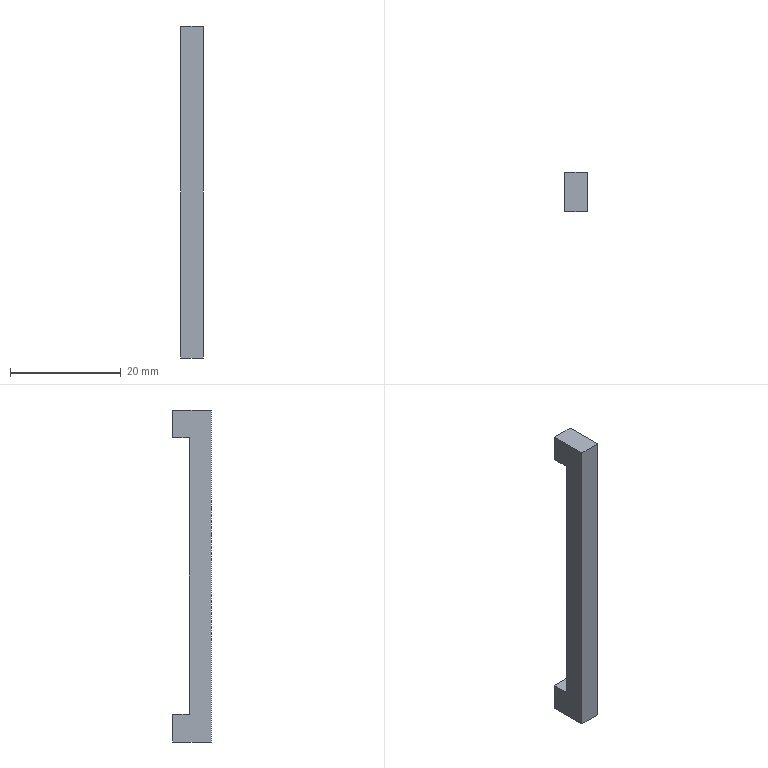Component | NX | KEY | 1 solid | 10 faces | box 4 x 7 x 60 mm | volume 1080 mm3 | plane 10
STEP:
#1=CARTESIAN_POINT('',(0.,0.,0.));
#2=DIRECTION('',(0.,0.,1.));
#3=DIRECTION('',(1.,0.,0.));
#4=AXIS2_PLACEMENT_3D('',#1,#2,#3);
#5=CARTESIAN_POINT('',(5.5,-11.365,13.5));
#6=VERTEX_POINT('',#5);
#7=CARTESIAN_POINT('',(5.5,-11.365,63.5));
#8=VERTEX_POINT('',#7);
#9=CARTESIAN_POINT('',(5.5,-11.365,38.5));
#10=DIRECTION('',(0.,0.,1.));
#11=VECTOR('',#10,1.);
#12=LINE('',#9,#11);
#13=CARTESIAN_POINT('',(9.5,-11.365,38.5));
#14=DIRECTION('',(0.,-1.,0.));
#15=DIRECTION('',(0.,-0.,-1.));
#16=AXIS2_PLACEMENT_3D('',#13,#14,#15);
#17=PLANE('',#16);
#18=CARTESIAN_POINT('',(0.,-4.));
#19=DIRECTION('',(-1.,0.));
#20=VECTOR('',#19,1.);
#21=LINE('',#18,#20);
#22=(GEOMETRIC_REPRESENTATION_CONTEXT(2)PARAMETRIC_REPRESENTATION_CONTEXT()REPRESENTATION_CONTEXT('',''));
#23=DEFINITIONAL_REPRESENTATION('',(#21),#22);
#24=PCURVE('',#17,#23);
#25=CARTESIAN_POINT('',(5.5,-11.365,38.5));
#26=DIRECTION('',(-1.,0.,0.));
#27=DIRECTION('',(0.,0.,1.));
#28=AXIS2_PLACEMENT_3D('',#25,#26,#27);
#29=PLANE('',#28);
#30=CARTESIAN_POINT('',(0.,0.));
#31=DIRECTION('',(1.,0.));
#32=VECTOR('',#31,1.);
#33=LINE('',#30,#32);
#34=(GEOMETRIC_REPRESENTATION_CONTEXT(2)PARAMETRIC_REPRESENTATION_CONTEXT()REPRESENTATION_CONTEXT('',''));
#35=DEFINITIONAL_REPRESENTATION('',(#33),#34);
#36=PCURVE('',#29,#35);
#37=SURFACE_CURVE('',#12,(#24,#36),.PCURVE_S1.);
#38=EDGE_CURVE('',#6,#8,#37,.T.);
#39=ORIENTED_EDGE('',*,*,#38,.T.);
#40=CARTESIAN_POINT('',(9.5,-11.365,63.5));
#41=VERTEX_POINT('',#40);
#42=CARTESIAN_POINT('',(9.5,-11.365,63.5));
#43=DIRECTION('',(-1.,0.,0.));
#44=VECTOR('',#43,1.);
#45=LINE('',#42,#44);
#46=CARTESIAN_POINT('',(-25.,0.));
#47=DIRECTION('',(0.,-1.));
#48=VECTOR('',#47,1.);
#49=LINE('',#46,#48);
#50=(GEOMETRIC_REPRESENTATION_CONTEXT(2)PARAMETRIC_REPRESENTATION_CONTEXT()REPRESENTATION_CONTEXT('',''));
#51=DEFINITIONAL_REPRESENTATION('',(#49),#50);
#52=PCURVE('',#17,#51);
#53=CARTESIAN_POINT('',(9.5,-11.365,63.5));
#54=DIRECTION('',(0.,0.,1.));
#55=DIRECTION('',(1.,0.,0.));
#56=AXIS2_PLACEMENT_3D('',#53,#54,#55);
#57=PLANE('',#56);
#58=CARTESIAN_POINT('',(0.,0.));
#59=DIRECTION('',(-1.,0.));
#60=VECTOR('',#59,1.);
#61=LINE('',#58,#60);
#62=(GEOMETRIC_REPRESENTATION_CONTEXT(2)PARAMETRIC_REPRESENTATION_CONTEXT()REPRESENTATION_CONTEXT('',''));
#63=DEFINITIONAL_REPRESENTATION('',(#61),#62);
#64=PCURVE('',#57,#63);
#65=SURFACE_CURVE('',#45,(#52,#64),.PCURVE_S1.);
#66=EDGE_CURVE('',#41,#8,#65,.T.);
#67=ORIENTED_EDGE('',*,*,#66,.F.);
#68=CARTESIAN_POINT('',(9.5,-11.365,13.5));
#69=VERTEX_POINT('',#68);
#70=CARTESIAN_POINT('',(9.5,-11.365,13.5));
#71=DIRECTION('',(0.,-0.,1.));
#72=VECTOR('',#71,1.);
#73=LINE('',#70,#72);
#74=CARTESIAN_POINT('',(25.,0.));
#75=DIRECTION('',(-1.,0.));
#76=VECTOR('',#75,1.);
#77=LINE('',#74,#76);
#78=(GEOMETRIC_REPRESENTATION_CONTEXT(2)PARAMETRIC_REPRESENTATION_CONTEXT()REPRESENTATION_CONTEXT('',''));
#79=DEFINITIONAL_REPRESENTATION('',(#77),#78);
#80=PCURVE('',#17,#79);
#81=CARTESIAN_POINT('',(9.5,-11.365,38.5));
#82=DIRECTION('',(-1.,0.,0.));
#83=DIRECTION('',(0.,0.,1.));
#84=AXIS2_PLACEMENT_3D('',#81,#82,#83);
#85=PLANE('',#84);
#86=CARTESIAN_POINT('',(-25.,0.));
#87=DIRECTION('',(1.,-0.));
#88=VECTOR('',#87,1.);
#89=LINE('',#86,#88);
#90=(GEOMETRIC_REPRESENTATION_CONTEXT(2)PARAMETRIC_REPRESENTATION_CONTEXT()REPRESENTATION_CONTEXT('',''));
#91=DEFINITIONAL_REPRESENTATION('',(#89),#90);
#92=PCURVE('',#85,#91);
#93=SURFACE_CURVE('',#73,(#80,#92),.PCURVE_S1.);
#94=EDGE_CURVE('',#69,#41,#93,.T.);
#95=ORIENTED_EDGE('',*,*,#94,.F.);
#96=CARTESIAN_POINT('',(9.5,-11.365,13.5));
#97=DIRECTION('',(-1.,0.,0.));
#98=VECTOR('',#97,1.);
#99=LINE('',#96,#98);
#100=CARTESIAN_POINT('',(25.,0.));
#101=DIRECTION('',(0.,-1.));
#102=VECTOR('',#101,1.);
#103=LINE('',#100,#102);
#104=(GEOMETRIC_REPRESENTATION_CONTEXT(2)PARAMETRIC_REPRESENTATION_CONTEXT()REPRESENTATION_CONTEXT('',''));
#105=DEFINITIONAL_REPRESENTATION('',(#103),#104);
#106=PCURVE('',#17,#105);
#107=CARTESIAN_POINT('',(9.5,-8.365,13.5));
#108=DIRECTION('',(0.,0.,-1.));
#109=DIRECTION('',(-1.,0.,0.));
#110=AXIS2_PLACEMENT_3D('',#107,#108,#109);
#111=PLANE('',#110);
#112=CARTESIAN_POINT('',(0.,-3.));
#113=DIRECTION('',(1.,0.));
#114=VECTOR('',#113,1.);
#115=LINE('',#112,#114);
#116=(GEOMETRIC_REPRESENTATION_CONTEXT(2)PARAMETRIC_REPRESENTATION_CONTEXT()REPRESENTATION_CONTEXT('',''));
#117=DEFINITIONAL_REPRESENTATION('',(#115),#116);
#118=PCURVE('',#111,#117);
#119=SURFACE_CURVE('',#99,(#106,#118),.PCURVE_S1.);
#120=EDGE_CURVE('',#69,#6,#119,.T.);
#121=ORIENTED_EDGE('',*,*,#120,.T.);
#122=EDGE_LOOP('',(#39,#67,#95,#121));
#123=FACE_BOUND('',#122,.T.);
#124=ADVANCED_FACE('',(#123),#17,.F.);
#125=CARTESIAN_POINT('',(5.5,-8.365,63.5));
#126=VERTEX_POINT('',#125);
#127=CARTESIAN_POINT('',(5.5,-11.365,63.5));
#128=DIRECTION('',(0.,1.,0.));
#129=VECTOR('',#128,1.);
#130=LINE('',#127,#129);
#131=CARTESIAN_POINT('',(-4.,0.));
#132=DIRECTION('',(0.,1.));
#133=VECTOR('',#132,1.);
#134=LINE('',#131,#133);
#135=(GEOMETRIC_REPRESENTATION_CONTEXT(2)PARAMETRIC_REPRESENTATION_CONTEXT()REPRESENTATION_CONTEXT('',''));
#136=DEFINITIONAL_REPRESENTATION('',(#134),#135);
#137=PCURVE('',#57,#136);
#138=CARTESIAN_POINT('',(25.,0.));
#139=DIRECTION('',(0.,1.));
#140=VECTOR('',#139,1.);
#141=LINE('',#138,#140);
#142=(GEOMETRIC_REPRESENTATION_CONTEXT(2)PARAMETRIC_REPRESENTATION_CONTEXT()REPRESENTATION_CONTEXT('',''));
#143=DEFINITIONAL_REPRESENTATION('',(#141),#142);
#144=PCURVE('',#29,#143);
#145=SURFACE_CURVE('',#130,(#137,#144),.PCURVE_S1.);
#146=EDGE_CURVE('',#8,#126,#145,.T.);
#147=ORIENTED_EDGE('',*,*,#146,.T.);
#148=CARTESIAN_POINT('',(9.5,-8.365,63.5));
#149=VERTEX_POINT('',#148);
#150=CARTESIAN_POINT('',(9.5,-8.365,63.5));
#151=DIRECTION('',(-1.,0.,0.));
#152=VECTOR('',#151,1.);
#153=LINE('',#150,#152);
#154=CARTESIAN_POINT('',(0.,3.));
#155=DIRECTION('',(-1.,0.));
#156=VECTOR('',#155,1.);
#157=LINE('',#154,#156);
#158=(GEOMETRIC_REPRESENTATION_CONTEXT(2)PARAMETRIC_REPRESENTATION_CONTEXT()REPRESENTATION_CONTEXT('',''));
#159=DEFINITIONAL_REPRESENTATION('',(#157),#158);
#160=PCURVE('',#57,#159);
#161=CARTESIAN_POINT('',(9.5,-8.365,63.5));
#162=DIRECTION('',(0.,-1.,0.));
#163=DIRECTION('',(0.,-0.,-1.));
#164=AXIS2_PLACEMENT_3D('',#161,#162,#163);
#165=PLANE('',#164);
#166=CARTESIAN_POINT('',(0.,0.));
#167=DIRECTION('',(0.,-1.));
#168=VECTOR('',#167,1.);
#169=LINE('',#166,#168);
#170=(GEOMETRIC_REPRESENTATION_CONTEXT(2)PARAMETRIC_REPRESENTATION_CONTEXT()REPRESENTATION_CONTEXT('',''));
#171=DEFINITIONAL_REPRESENTATION('',(#169),#170);
#172=PCURVE('',#165,#171);
#173=SURFACE_CURVE('',#153,(#160,#172),.PCURVE_S1.);
#174=EDGE_CURVE('',#149,#126,#173,.T.);
#175=ORIENTED_EDGE('',*,*,#174,.F.);
#176=CARTESIAN_POINT('',(9.5,-11.365,63.5));
#177=DIRECTION('',(0.,1.,0.));
#178=VECTOR('',#177,1.);
#179=LINE('',#176,#178);
#180=CARTESIAN_POINT('',(0.,0.));
#181=DIRECTION('',(0.,1.));
#182=VECTOR('',#181,1.);
#183=LINE('',#180,#182);
#184=(GEOMETRIC_REPRESENTATION_CONTEXT(2)PARAMETRIC_REPRESENTATION_CONTEXT()REPRESENTATION_CONTEXT('',''));
#185=DEFINITIONAL_REPRESENTATION('',(#183),#184);
#186=PCURVE('',#57,#185);
#187=CARTESIAN_POINT('',(25.,0.));
#188=DIRECTION('',(0.,1.));
#189=VECTOR('',#188,1.);
#190=LINE('',#187,#189);
#191=(GEOMETRIC_REPRESENTATION_CONTEXT(2)PARAMETRIC_REPRESENTATION_CONTEXT()REPRESENTATION_CONTEXT('',''));
#192=DEFINITIONAL_REPRESENTATION('',(#190),#191);
#193=PCURVE('',#85,#192);
#194=SURFACE_CURVE('',#179,(#186,#193),.PCURVE_S1.);
#195=EDGE_CURVE('',#41,#149,#194,.T.);
#196=ORIENTED_EDGE('',*,*,#195,.F.);
#197=ORIENTED_EDGE('',*,*,#66,.T.);
#198=EDGE_LOOP('',(#147,#175,#196,#197));
#199=FACE_BOUND('',#198,.T.);
#200=ADVANCED_FACE('',(#199),#57,.F.);
#201=CARTESIAN_POINT('',(5.5,-8.365,68.5));
#202=VERTEX_POINT('',#201);
#203=CARTESIAN_POINT('',(5.5,-8.365,63.5));
#204=DIRECTION('',(0.,0.,1.));
#205=VECTOR('',#204,1.);
#206=LINE('',#203,#205);
#207=CARTESIAN_POINT('',(0.,-4.));
#208=DIRECTION('',(-1.,0.));
#209=VECTOR('',#208,1.);
#210=LINE('',#207,#209);
#211=(GEOMETRIC_REPRESENTATION_CONTEXT(2)PARAMETRIC_REPRESENTATION_CONTEXT()REPRESENTATION_CONTEXT('',''));
#212=DEFINITIONAL_REPRESENTATION('',(#210),#211);
#213=PCURVE('',#165,#212);
#214=CARTESIAN_POINT('',(25.,3.));
#215=DIRECTION('',(1.,0.));
#216=VECTOR('',#215,1.);
#217=LINE('',#214,#216);
#218=(GEOMETRIC_REPRESENTATION_CONTEXT(2)PARAMETRIC_REPRESENTATION_CONTEXT()REPRESENTATION_CONTEXT('',''));
#219=DEFINITIONAL_REPRESENTATION('',(#217),#218);
#220=PCURVE('',#29,#219);
#221=SURFACE_CURVE('',#206,(#213,#220),.PCURVE_S1.);
#222=EDGE_CURVE('',#126,#202,#221,.T.);
#223=ORIENTED_EDGE('',*,*,#222,.T.);
#224=CARTESIAN_POINT('',(9.5,-8.365,68.5));
#225=VERTEX_POINT('',#224);
#226=CARTESIAN_POINT('',(9.5,-8.365,68.5));
#227=DIRECTION('',(-1.,0.,0.));
#228=VECTOR('',#227,1.);
#229=LINE('',#226,#228);
#230=CARTESIAN_POINT('',(-5.,0.));
#231=DIRECTION('',(0.,-1.));
#232=VECTOR('',#231,1.);
#233=LINE('',#230,#232);
#234=(GEOMETRIC_REPRESENTATION_CONTEXT(2)PARAMETRIC_REPRESENTATION_CONTEXT()REPRESENTATION_CONTEXT('',''));
#235=DEFINITIONAL_REPRESENTATION('',(#233),#234);
#236=PCURVE('',#165,#235);
#237=CARTESIAN_POINT('',(9.5,-8.365,68.5));
#238=DIRECTION('',(0.,0.,-1.));
#239=DIRECTION('',(-1.,0.,0.));
#240=AXIS2_PLACEMENT_3D('',#237,#238,#239);
#241=PLANE('',#240);
#242=CARTESIAN_POINT('',(0.,0.));
#243=DIRECTION('',(1.,0.));
#244=VECTOR('',#243,1.);
#245=LINE('',#242,#244);
#246=(GEOMETRIC_REPRESENTATION_CONTEXT(2)PARAMETRIC_REPRESENTATION_CONTEXT()REPRESENTATION_CONTEXT('',''));
#247=DEFINITIONAL_REPRESENTATION('',(#245),#246);
#248=PCURVE('',#241,#247);
#249=SURFACE_CURVE('',#229,(#236,#248),.PCURVE_S1.);
#250=EDGE_CURVE('',#225,#202,#249,.T.);
#251=ORIENTED_EDGE('',*,*,#250,.F.);
#252=CARTESIAN_POINT('',(9.5,-8.365,63.5));
#253=DIRECTION('',(0.,0.,1.));
#254=VECTOR('',#253,1.);
#255=LINE('',#252,#254);
#256=CARTESIAN_POINT('',(0.,0.));
#257=DIRECTION('',(-1.,0.));
#258=VECTOR('',#257,1.);
#259=LINE('',#256,#258);
#260=(GEOMETRIC_REPRESENTATION_CONTEXT(2)PARAMETRIC_REPRESENTATION_CONTEXT()REPRESENTATION_CONTEXT('',''));
#261=DEFINITIONAL_REPRESENTATION('',(#259),#260);
#262=PCURVE('',#165,#261);
#263=CARTESIAN_POINT('',(25.,3.));
#264=DIRECTION('',(1.,0.));
#265=VECTOR('',#264,1.);
#266=LINE('',#263,#265);
#267=(GEOMETRIC_REPRESENTATION_CONTEXT(2)PARAMETRIC_REPRESENTATION_CONTEXT()REPRESENTATION_CONTEXT('',''));
#268=DEFINITIONAL_REPRESENTATION('',(#266),#267);
#269=PCURVE('',#85,#268);
#270=SURFACE_CURVE('',#255,(#262,#269),.PCURVE_S1.);
#271=EDGE_CURVE('',#149,#225,#270,.T.);
#272=ORIENTED_EDGE('',*,*,#271,.F.);
#273=ORIENTED_EDGE('',*,*,#174,.T.);
#274=EDGE_LOOP('',(#223,#251,#272,#273));
#275=FACE_BOUND('',#274,.T.);
#276=ADVANCED_FACE('',(#275),#165,.F.);
#277=CARTESIAN_POINT('',(5.5,-15.365,68.5));
#278=VERTEX_POINT('',#277);
#279=CARTESIAN_POINT('',(5.5,-8.365,68.5));
#280=DIRECTION('',(0.,-1.,0.));
#281=VECTOR('',#280,1.);
#282=LINE('',#279,#281);
#283=CARTESIAN_POINT('',(4.,0.));
#284=DIRECTION('',(0.,-1.));
#285=VECTOR('',#284,1.);
#286=LINE('',#283,#285);
#287=(GEOMETRIC_REPRESENTATION_CONTEXT(2)PARAMETRIC_REPRESENTATION_CONTEXT()REPRESENTATION_CONTEXT('',''));
#288=DEFINITIONAL_REPRESENTATION('',(#286),#287);
#289=PCURVE('',#241,#288);
#290=CARTESIAN_POINT('',(30.,3.));
#291=DIRECTION('',(0.,-1.));
#292=VECTOR('',#291,1.);
#293=LINE('',#290,#292);
#294=(GEOMETRIC_REPRESENTATION_CONTEXT(2)PARAMETRIC_REPRESENTATION_CONTEXT()REPRESENTATION_CONTEXT('',''));
#295=DEFINITIONAL_REPRESENTATION('',(#293),#294);
#296=PCURVE('',#29,#295);
#297=SURFACE_CURVE('',#282,(#289,#296),.PCURVE_S1.);
#298=EDGE_CURVE('',#202,#278,#297,.T.);
#299=ORIENTED_EDGE('',*,*,#298,.T.);
#300=CARTESIAN_POINT('',(9.5,-15.365,68.5));
#301=VERTEX_POINT('',#300);
#302=CARTESIAN_POINT('',(9.5,-15.365,68.5));
#303=DIRECTION('',(-1.,0.,0.));
#304=VECTOR('',#303,1.);
#305=LINE('',#302,#304);
#306=CARTESIAN_POINT('',(0.,-7.));
#307=DIRECTION('',(1.,0.));
#308=VECTOR('',#307,1.);
#309=LINE('',#306,#308);
#310=(GEOMETRIC_REPRESENTATION_CONTEXT(2)PARAMETRIC_REPRESENTATION_CONTEXT()REPRESENTATION_CONTEXT('',''));
#311=DEFINITIONAL_REPRESENTATION('',(#309),#310);
#312=PCURVE('',#241,#311);
#313=CARTESIAN_POINT('',(9.5,-15.365,38.5));
#314=DIRECTION('',(0.,1.,0.));
#315=DIRECTION('',(0.,-0.,1.));
#316=AXIS2_PLACEMENT_3D('',#313,#314,#315);
#317=PLANE('',#316);
#318=CARTESIAN_POINT('',(30.,0.));
#319=DIRECTION('',(0.,-1.));
#320=VECTOR('',#319,1.);
#321=LINE('',#318,#320);
#322=(GEOMETRIC_REPRESENTATION_CONTEXT(2)PARAMETRIC_REPRESENTATION_CONTEXT()REPRESENTATION_CONTEXT('',''));
#323=DEFINITIONAL_REPRESENTATION('',(#321),#322);
#324=PCURVE('',#317,#323);
#325=SURFACE_CURVE('',#305,(#312,#324),.PCURVE_S1.);
#326=EDGE_CURVE('',#301,#278,#325,.T.);
#327=ORIENTED_EDGE('',*,*,#326,.F.);
#328=CARTESIAN_POINT('',(9.5,-8.365,68.5));
#329=DIRECTION('',(0.,-1.,0.));
#330=VECTOR('',#329,1.);
#331=LINE('',#328,#330);
#332=CARTESIAN_POINT('',(0.,0.));
#333=DIRECTION('',(0.,-1.));
#334=VECTOR('',#333,1.);
#335=LINE('',#332,#334);
#336=(GEOMETRIC_REPRESENTATION_CONTEXT(2)PARAMETRIC_REPRESENTATION_CONTEXT()REPRESENTATION_CONTEXT('',''));
#337=DEFINITIONAL_REPRESENTATION('',(#335),#336);
#338=PCURVE('',#241,#337);
#339=CARTESIAN_POINT('',(30.,3.));
#340=DIRECTION('',(0.,-1.));
#341=VECTOR('',#340,1.);
#342=LINE('',#339,#341);
#343=(GEOMETRIC_REPRESENTATION_CONTEXT(2)PARAMETRIC_REPRESENTATION_CONTEXT()REPRESENTATION_CONTEXT('',''));
#344=DEFINITIONAL_REPRESENTATION('',(#342),#343);
#345=PCURVE('',#85,#344);
#346=SURFACE_CURVE('',#331,(#338,#345),.PCURVE_S1.);
#347=EDGE_CURVE('',#225,#301,#346,.T.);
#348=ORIENTED_EDGE('',*,*,#347,.F.);
#349=ORIENTED_EDGE('',*,*,#250,.T.);
#350=EDGE_LOOP('',(#299,#327,#348,#349));
#351=FACE_BOUND('',#350,.T.);
#352=ADVANCED_FACE('',(#351),#241,.F.);
#353=CARTESIAN_POINT('',(5.5,-15.365,8.5));
#354=VERTEX_POINT('',#353);
#355=CARTESIAN_POINT('',(5.5,-15.365,38.5));
#356=DIRECTION('',(0.,0.,-1.));
#357=VECTOR('',#356,1.);
#358=LINE('',#355,#357);
#359=CARTESIAN_POINT('',(0.,-4.));
#360=DIRECTION('',(-1.,0.));
#361=VECTOR('',#360,1.);
#362=LINE('',#359,#361);
#363=(GEOMETRIC_REPRESENTATION_CONTEXT(2)PARAMETRIC_REPRESENTATION_CONTEXT()REPRESENTATION_CONTEXT('',''));
#364=DEFINITIONAL_REPRESENTATION('',(#362),#363);
#365=PCURVE('',#317,#364);
#366=CARTESIAN_POINT('',(0.,-4.));
#367=DIRECTION('',(-1.,0.));
#368=VECTOR('',#367,1.);
#369=LINE('',#366,#368);
#370=(GEOMETRIC_REPRESENTATION_CONTEXT(2)PARAMETRIC_REPRESENTATION_CONTEXT()REPRESENTATION_CONTEXT('',''));
#371=DEFINITIONAL_REPRESENTATION('',(#369),#370);
#372=PCURVE('',#29,#371);
#373=SURFACE_CURVE('',#358,(#365,#372),.PCURVE_S1.);
#374=EDGE_CURVE('',#278,#354,#373,.T.);
#375=ORIENTED_EDGE('',*,*,#374,.T.);
#376=CARTESIAN_POINT('',(9.5,-15.365,8.5));
#377=VERTEX_POINT('',#376);
#378=CARTESIAN_POINT('',(9.5,-15.365,8.5));
#379=DIRECTION('',(-1.,0.,0.));
#380=VECTOR('',#379,1.);
#381=LINE('',#378,#380);
#382=CARTESIAN_POINT('',(-30.,0.));
#383=DIRECTION('',(0.,-1.));
#384=VECTOR('',#383,1.);
#385=LINE('',#382,#384);
#386=(GEOMETRIC_REPRESENTATION_CONTEXT(2)PARAMETRIC_REPRESENTATION_CONTEXT()REPRESENTATION_CONTEXT('',''));
#387=DEFINITIONAL_REPRESENTATION('',(#385),#386);
#388=PCURVE('',#317,#387);
#389=CARTESIAN_POINT('',(9.5,-15.365,8.5));
#390=DIRECTION('',(0.,0.,1.));
#391=DIRECTION('',(1.,0.,0.));
#392=AXIS2_PLACEMENT_3D('',#389,#390,#391);
#393=PLANE('',#392);
#394=CARTESIAN_POINT('',(0.,0.));
#395=DIRECTION('',(-1.,0.));
#396=VECTOR('',#395,1.);
#397=LINE('',#394,#396);
#398=(GEOMETRIC_REPRESENTATION_CONTEXT(2)PARAMETRIC_REPRESENTATION_CONTEXT()REPRESENTATION_CONTEXT('',''));
#399=DEFINITIONAL_REPRESENTATION('',(#397),#398);
#400=PCURVE('',#393,#399);
#401=SURFACE_CURVE('',#381,(#388,#400),.PCURVE_S1.);
#402=EDGE_CURVE('',#377,#354,#401,.T.);
#403=ORIENTED_EDGE('',*,*,#402,.F.);
#404=CARTESIAN_POINT('',(9.5,-15.365,68.5));
#405=DIRECTION('',(0.,-0.,-1.));
#406=VECTOR('',#405,1.);
#407=LINE('',#404,#406);
#408=CARTESIAN_POINT('',(30.,0.));
#409=DIRECTION('',(-1.,0.));
#410=VECTOR('',#409,1.);
#411=LINE('',#408,#410);
#412=(GEOMETRIC_REPRESENTATION_CONTEXT(2)PARAMETRIC_REPRESENTATION_CONTEXT()REPRESENTATION_CONTEXT('',''));
#413=DEFINITIONAL_REPRESENTATION('',(#411),#412);
#414=PCURVE('',#317,#413);
#415=CARTESIAN_POINT('',(30.,-4.));
#416=DIRECTION('',(-1.,-0.));
#417=VECTOR('',#416,1.);
#418=LINE('',#415,#417);
#419=(GEOMETRIC_REPRESENTATION_CONTEXT(2)PARAMETRIC_REPRESENTATION_CONTEXT()REPRESENTATION_CONTEXT('',''));
#420=DEFINITIONAL_REPRESENTATION('',(#418),#419);
#421=PCURVE('',#85,#420);
#422=SURFACE_CURVE('',#407,(#414,#421),.PCURVE_S1.);
#423=EDGE_CURVE('',#301,#377,#422,.T.);
#424=ORIENTED_EDGE('',*,*,#423,.F.);
#425=ORIENTED_EDGE('',*,*,#326,.T.);
#426=EDGE_LOOP('',(#375,#403,#424,#425));
#427=FACE_BOUND('',#426,.T.);
#428=ADVANCED_FACE('',(#427),#317,.F.);
#429=CARTESIAN_POINT('',(5.5,-8.365,8.5));
#430=VERTEX_POINT('',#429);
#431=CARTESIAN_POINT('',(5.5,-15.365,8.5));
#432=DIRECTION('',(0.,1.,0.));
#433=VECTOR('',#432,1.);
#434=LINE('',#431,#433);
#435=CARTESIAN_POINT('',(-4.,0.));
#436=DIRECTION('',(0.,1.));
#437=VECTOR('',#436,1.);
#438=LINE('',#435,#437);
#439=(GEOMETRIC_REPRESENTATION_CONTEXT(2)PARAMETRIC_REPRESENTATION_CONTEXT()REPRESENTATION_CONTEXT('',''));
#440=DEFINITIONAL_REPRESENTATION('',(#438),#439);
#441=PCURVE('',#393,#440);
#442=CARTESIAN_POINT('',(-30.,-4.));
#443=DIRECTION('',(0.,1.));
#444=VECTOR('',#443,1.);
#445=LINE('',#442,#444);
#446=(GEOMETRIC_REPRESENTATION_CONTEXT(2)PARAMETRIC_REPRESENTATION_CONTEXT()REPRESENTATION_CONTEXT('',''));
#447=DEFINITIONAL_REPRESENTATION('',(#445),#446);
#448=PCURVE('',#29,#447);
#449=SURFACE_CURVE('',#434,(#441,#448),.PCURVE_S1.);
#450=EDGE_CURVE('',#354,#430,#449,.T.);
#451=ORIENTED_EDGE('',*,*,#450,.T.);
#452=CARTESIAN_POINT('',(9.5,-8.365,8.5));
#453=VERTEX_POINT('',#452);
#454=CARTESIAN_POINT('',(9.5,-8.365,8.5));
#455=DIRECTION('',(-1.,0.,0.));
#456=VECTOR('',#455,1.);
#457=LINE('',#454,#456);
#458=CARTESIAN_POINT('',(0.,7.));
#459=DIRECTION('',(-1.,0.));
#460=VECTOR('',#459,1.);
#461=LINE('',#458,#460);
#462=(GEOMETRIC_REPRESENTATION_CONTEXT(2)PARAMETRIC_REPRESENTATION_CONTEXT()REPRESENTATION_CONTEXT('',''));
#463=DEFINITIONAL_REPRESENTATION('',(#461),#462);
#464=PCURVE('',#393,#463);
#465=CARTESIAN_POINT('',(9.5,-8.365,8.5));
#466=DIRECTION('',(0.,-1.,-0.));
#467=DIRECTION('',(0.,0.,-1.));
#468=AXIS2_PLACEMENT_3D('',#465,#466,#467);
#469=PLANE('',#468);
#470=CARTESIAN_POINT('',(0.,0.));
#471=DIRECTION('',(0.,-1.));
#472=VECTOR('',#471,1.);
#473=LINE('',#470,#472);
#474=(GEOMETRIC_REPRESENTATION_CONTEXT(2)PARAMETRIC_REPRESENTATION_CONTEXT()REPRESENTATION_CONTEXT('',''));
#475=DEFINITIONAL_REPRESENTATION('',(#473),#474);
#476=PCURVE('',#469,#475);
#477=SURFACE_CURVE('',#457,(#464,#476),.PCURVE_S1.);
#478=EDGE_CURVE('',#453,#430,#477,.T.);
#479=ORIENTED_EDGE('',*,*,#478,.F.);
#480=CARTESIAN_POINT('',(9.5,-15.365,8.5));
#481=DIRECTION('',(0.,1.,0.));
#482=VECTOR('',#481,1.);
#483=LINE('',#480,#482);
#484=CARTESIAN_POINT('',(0.,0.));
#485=DIRECTION('',(0.,1.));
#486=VECTOR('',#485,1.);
#487=LINE('',#484,#486);
#488=(GEOMETRIC_REPRESENTATION_CONTEXT(2)PARAMETRIC_REPRESENTATION_CONTEXT()REPRESENTATION_CONTEXT('',''));
#489=DEFINITIONAL_REPRESENTATION('',(#487),#488);
#490=PCURVE('',#393,#489);
#491=CARTESIAN_POINT('',(-30.,-4.));
#492=DIRECTION('',(0.,1.));
#493=VECTOR('',#492,1.);
#494=LINE('',#491,#493);
#495=(GEOMETRIC_REPRESENTATION_CONTEXT(2)PARAMETRIC_REPRESENTATION_CONTEXT()REPRESENTATION_CONTEXT('',''));
#496=DEFINITIONAL_REPRESENTATION('',(#494),#495);
#497=PCURVE('',#85,#496);
#498=SURFACE_CURVE('',#483,(#490,#497),.PCURVE_S1.);
#499=EDGE_CURVE('',#377,#453,#498,.T.);
#500=ORIENTED_EDGE('',*,*,#499,.F.);
#501=ORIENTED_EDGE('',*,*,#402,.T.);
#502=EDGE_LOOP('',(#451,#479,#500,#501));
#503=FACE_BOUND('',#502,.T.);
#504=ADVANCED_FACE('',(#503),#393,.F.);
#505=CARTESIAN_POINT('',(5.5,-8.365,13.5));
#506=VERTEX_POINT('',#505);
#507=CARTESIAN_POINT('',(5.5,-8.365,8.5));
#508=DIRECTION('',(0.,-0.,1.));
#509=VECTOR('',#508,1.);
#510=LINE('',#507,#509);
#511=CARTESIAN_POINT('',(0.,-4.));
#512=DIRECTION('',(-1.,0.));
#513=VECTOR('',#512,1.);
#514=LINE('',#511,#513);
#515=(GEOMETRIC_REPRESENTATION_CONTEXT(2)PARAMETRIC_REPRESENTATION_CONTEXT()REPRESENTATION_CONTEXT('',''));
#516=DEFINITIONAL_REPRESENTATION('',(#514),#515);
#517=PCURVE('',#469,#516);
#518=CARTESIAN_POINT('',(-30.,3.));
#519=DIRECTION('',(1.,-0.));
#520=VECTOR('',#519,1.);
#521=LINE('',#518,#520);
#522=(GEOMETRIC_REPRESENTATION_CONTEXT(2)PARAMETRIC_REPRESENTATION_CONTEXT()REPRESENTATION_CONTEXT('',''));
#523=DEFINITIONAL_REPRESENTATION('',(#521),#522);
#524=PCURVE('',#29,#523);
#525=SURFACE_CURVE('',#510,(#517,#524),.PCURVE_S1.);
#526=EDGE_CURVE('',#430,#506,#525,.T.);
#527=ORIENTED_EDGE('',*,*,#526,.T.);
#528=CARTESIAN_POINT('',(9.5,-8.365,13.5));
#529=VERTEX_POINT('',#528);
#530=CARTESIAN_POINT('',(9.5,-8.365,13.5));
#531=DIRECTION('',(-1.,0.,0.));
#532=VECTOR('',#531,1.);
#533=LINE('',#530,#532);
#534=CARTESIAN_POINT('',(-5.,0.));
#535=DIRECTION('',(0.,-1.));
#536=VECTOR('',#535,1.);
#537=LINE('',#534,#536);
#538=(GEOMETRIC_REPRESENTATION_CONTEXT(2)PARAMETRIC_REPRESENTATION_CONTEXT()REPRESENTATION_CONTEXT('',''));
#539=DEFINITIONAL_REPRESENTATION('',(#537),#538);
#540=PCURVE('',#469,#539);
#541=CARTESIAN_POINT('',(0.,0.));
#542=DIRECTION('',(1.,0.));
#543=VECTOR('',#542,1.);
#544=LINE('',#541,#543);
#545=(GEOMETRIC_REPRESENTATION_CONTEXT(2)PARAMETRIC_REPRESENTATION_CONTEXT()REPRESENTATION_CONTEXT('',''));
#546=DEFINITIONAL_REPRESENTATION('',(#544),#545);
#547=PCURVE('',#111,#546);
#548=SURFACE_CURVE('',#533,(#540,#547),.PCURVE_S1.);
#549=EDGE_CURVE('',#529,#506,#548,.T.);
#550=ORIENTED_EDGE('',*,*,#549,.F.);
#551=CARTESIAN_POINT('',(9.5,-8.365,8.5));
#552=DIRECTION('',(0.,-0.,1.));
#553=VECTOR('',#552,1.);
#554=LINE('',#551,#553);
#555=CARTESIAN_POINT('',(0.,0.));
#556=DIRECTION('',(-1.,0.));
#557=VECTOR('',#556,1.);
#558=LINE('',#555,#557);
#559=(GEOMETRIC_REPRESENTATION_CONTEXT(2)PARAMETRIC_REPRESENTATION_CONTEXT()REPRESENTATION_CONTEXT('',''));
#560=DEFINITIONAL_REPRESENTATION('',(#558),#559);
#561=PCURVE('',#469,#560);
#562=CARTESIAN_POINT('',(-30.,3.));
#563=DIRECTION('',(1.,-0.));
#564=VECTOR('',#563,1.);
#565=LINE('',#562,#564);
#566=(GEOMETRIC_REPRESENTATION_CONTEXT(2)PARAMETRIC_REPRESENTATION_CONTEXT()REPRESENTATION_CONTEXT('',''));
#567=DEFINITIONAL_REPRESENTATION('',(#565),#566);
#568=PCURVE('',#85,#567);
#569=SURFACE_CURVE('',#554,(#561,#568),.PCURVE_S1.);
#570=EDGE_CURVE('',#453,#529,#569,.T.);
#571=ORIENTED_EDGE('',*,*,#570,.F.);
#572=ORIENTED_EDGE('',*,*,#478,.T.);
#573=EDGE_LOOP('',(#527,#550,#571,#572));
#574=FACE_BOUND('',#573,.T.);
#575=ADVANCED_FACE('',(#574),#469,.F.);
#576=CARTESIAN_POINT('',(5.5,-8.365,13.5));
#577=DIRECTION('',(0.,-1.,0.));
#578=VECTOR('',#577,1.);
#579=LINE('',#576,#578);
#580=CARTESIAN_POINT('',(4.,0.));
#581=DIRECTION('',(0.,-1.));
#582=VECTOR('',#581,1.);
#583=LINE('',#580,#582);
#584=(GEOMETRIC_REPRESENTATION_CONTEXT(2)PARAMETRIC_REPRESENTATION_CONTEXT()REPRESENTATION_CONTEXT('',''));
#585=DEFINITIONAL_REPRESENTATION('',(#583),#584);
#586=PCURVE('',#111,#585);
#587=CARTESIAN_POINT('',(-25.,3.));
#588=DIRECTION('',(0.,-1.));
#589=VECTOR('',#588,1.);
#590=LINE('',#587,#589);
#591=(GEOMETRIC_REPRESENTATION_CONTEXT(2)PARAMETRIC_REPRESENTATION_CONTEXT()REPRESENTATION_CONTEXT('',''));
#592=DEFINITIONAL_REPRESENTATION('',(#590),#591);
#593=PCURVE('',#29,#592);
#594=SURFACE_CURVE('',#579,(#586,#593),.PCURVE_S1.);
#595=EDGE_CURVE('',#506,#6,#594,.T.);
#596=ORIENTED_EDGE('',*,*,#595,.T.);
#597=ORIENTED_EDGE('',*,*,#120,.F.);
#598=CARTESIAN_POINT('',(9.5,-8.365,13.5));
#599=DIRECTION('',(0.,-1.,0.));
#600=VECTOR('',#599,1.);
#601=LINE('',#598,#600);
#602=CARTESIAN_POINT('',(0.,0.));
#603=DIRECTION('',(0.,-1.));
#604=VECTOR('',#603,1.);
#605=LINE('',#602,#604);
#606=(GEOMETRIC_REPRESENTATION_CONTEXT(2)PARAMETRIC_REPRESENTATION_CONTEXT()REPRESENTATION_CONTEXT('',''));
#607=DEFINITIONAL_REPRESENTATION('',(#605),#606);
#608=PCURVE('',#111,#607);
#609=CARTESIAN_POINT('',(-25.,3.));
#610=DIRECTION('',(0.,-1.));
#611=VECTOR('',#610,1.);
#612=LINE('',#609,#611);
#613=(GEOMETRIC_REPRESENTATION_CONTEXT(2)PARAMETRIC_REPRESENTATION_CONTEXT()REPRESENTATION_CONTEXT('',''));
#614=DEFINITIONAL_REPRESENTATION('',(#612),#613);
#615=PCURVE('',#85,#614);
#616=SURFACE_CURVE('',#601,(#608,#615),.PCURVE_S1.);
#617=EDGE_CURVE('',#529,#69,#616,.T.);
#618=ORIENTED_EDGE('',*,*,#617,.F.);
#619=ORIENTED_EDGE('',*,*,#549,.T.);
#620=EDGE_LOOP('',(#596,#597,#618,#619));
#621=FACE_BOUND('',#620,.T.);
#622=ADVANCED_FACE('',(#621),#111,.F.);
#623=ORIENTED_EDGE('',*,*,#94,.T.);
#624=ORIENTED_EDGE('',*,*,#195,.T.);
#625=ORIENTED_EDGE('',*,*,#271,.T.);
#626=ORIENTED_EDGE('',*,*,#347,.T.);
#627=ORIENTED_EDGE('',*,*,#423,.T.);
#628=ORIENTED_EDGE('',*,*,#499,.T.);
#629=ORIENTED_EDGE('',*,*,#570,.T.);
#630=ORIENTED_EDGE('',*,*,#617,.T.);
#631=EDGE_LOOP('',(#623,#624,#625,#626,#627,#628,#629,#630));
#632=FACE_BOUND('',#631,.T.);
#633=ADVANCED_FACE('',(#632),#85,.F.);
#634=ORIENTED_EDGE('',*,*,#38,.F.);
#635=ORIENTED_EDGE('',*,*,#595,.F.);
#636=ORIENTED_EDGE('',*,*,#526,.F.);
#637=ORIENTED_EDGE('',*,*,#450,.F.);
#638=ORIENTED_EDGE('',*,*,#374,.F.);
#639=ORIENTED_EDGE('',*,*,#298,.F.);
#640=ORIENTED_EDGE('',*,*,#222,.F.);
#641=ORIENTED_EDGE('',*,*,#146,.F.);
#642=EDGE_LOOP('',(#634,#635,#636,#637,#638,#639,#640,#641));
#643=FACE_BOUND('',#642,.T.);
#644=ADVANCED_FACE('',(#643),#29,.T.);
#645=CLOSED_SHELL('',(#124,#200,#276,#352,#428,#504,#575,#622,#633,#644));
#646=MANIFOLD_SOLID_BREP('',#645);
#647=(LENGTH_UNIT()NAMED_UNIT(*)SI_UNIT(.MILLI.,.METRE.));
#648=UNCERTAINTY_MEASURE_WITH_UNIT(LENGTH_MEASURE(0.0000001),#647,'','');
#649=(NAMED_UNIT(*)PLANE_ANGLE_UNIT()SI_UNIT($,.RADIAN.));
#650=(NAMED_UNIT(*)SI_UNIT($,.STERADIAN.)SOLID_ANGLE_UNIT());
#651=(GEOMETRIC_REPRESENTATION_CONTEXT(3)GLOBAL_UNCERTAINTY_ASSIGNED_CONTEXT((#648))GLOBAL_UNIT_ASSIGNED_CONTEXT((#647,#649,#650))REPRESENTATION_CONTEXT('',''));
#652=ADVANCED_BREP_SHAPE_REPRESENTATION('',(#4,#646),#651);